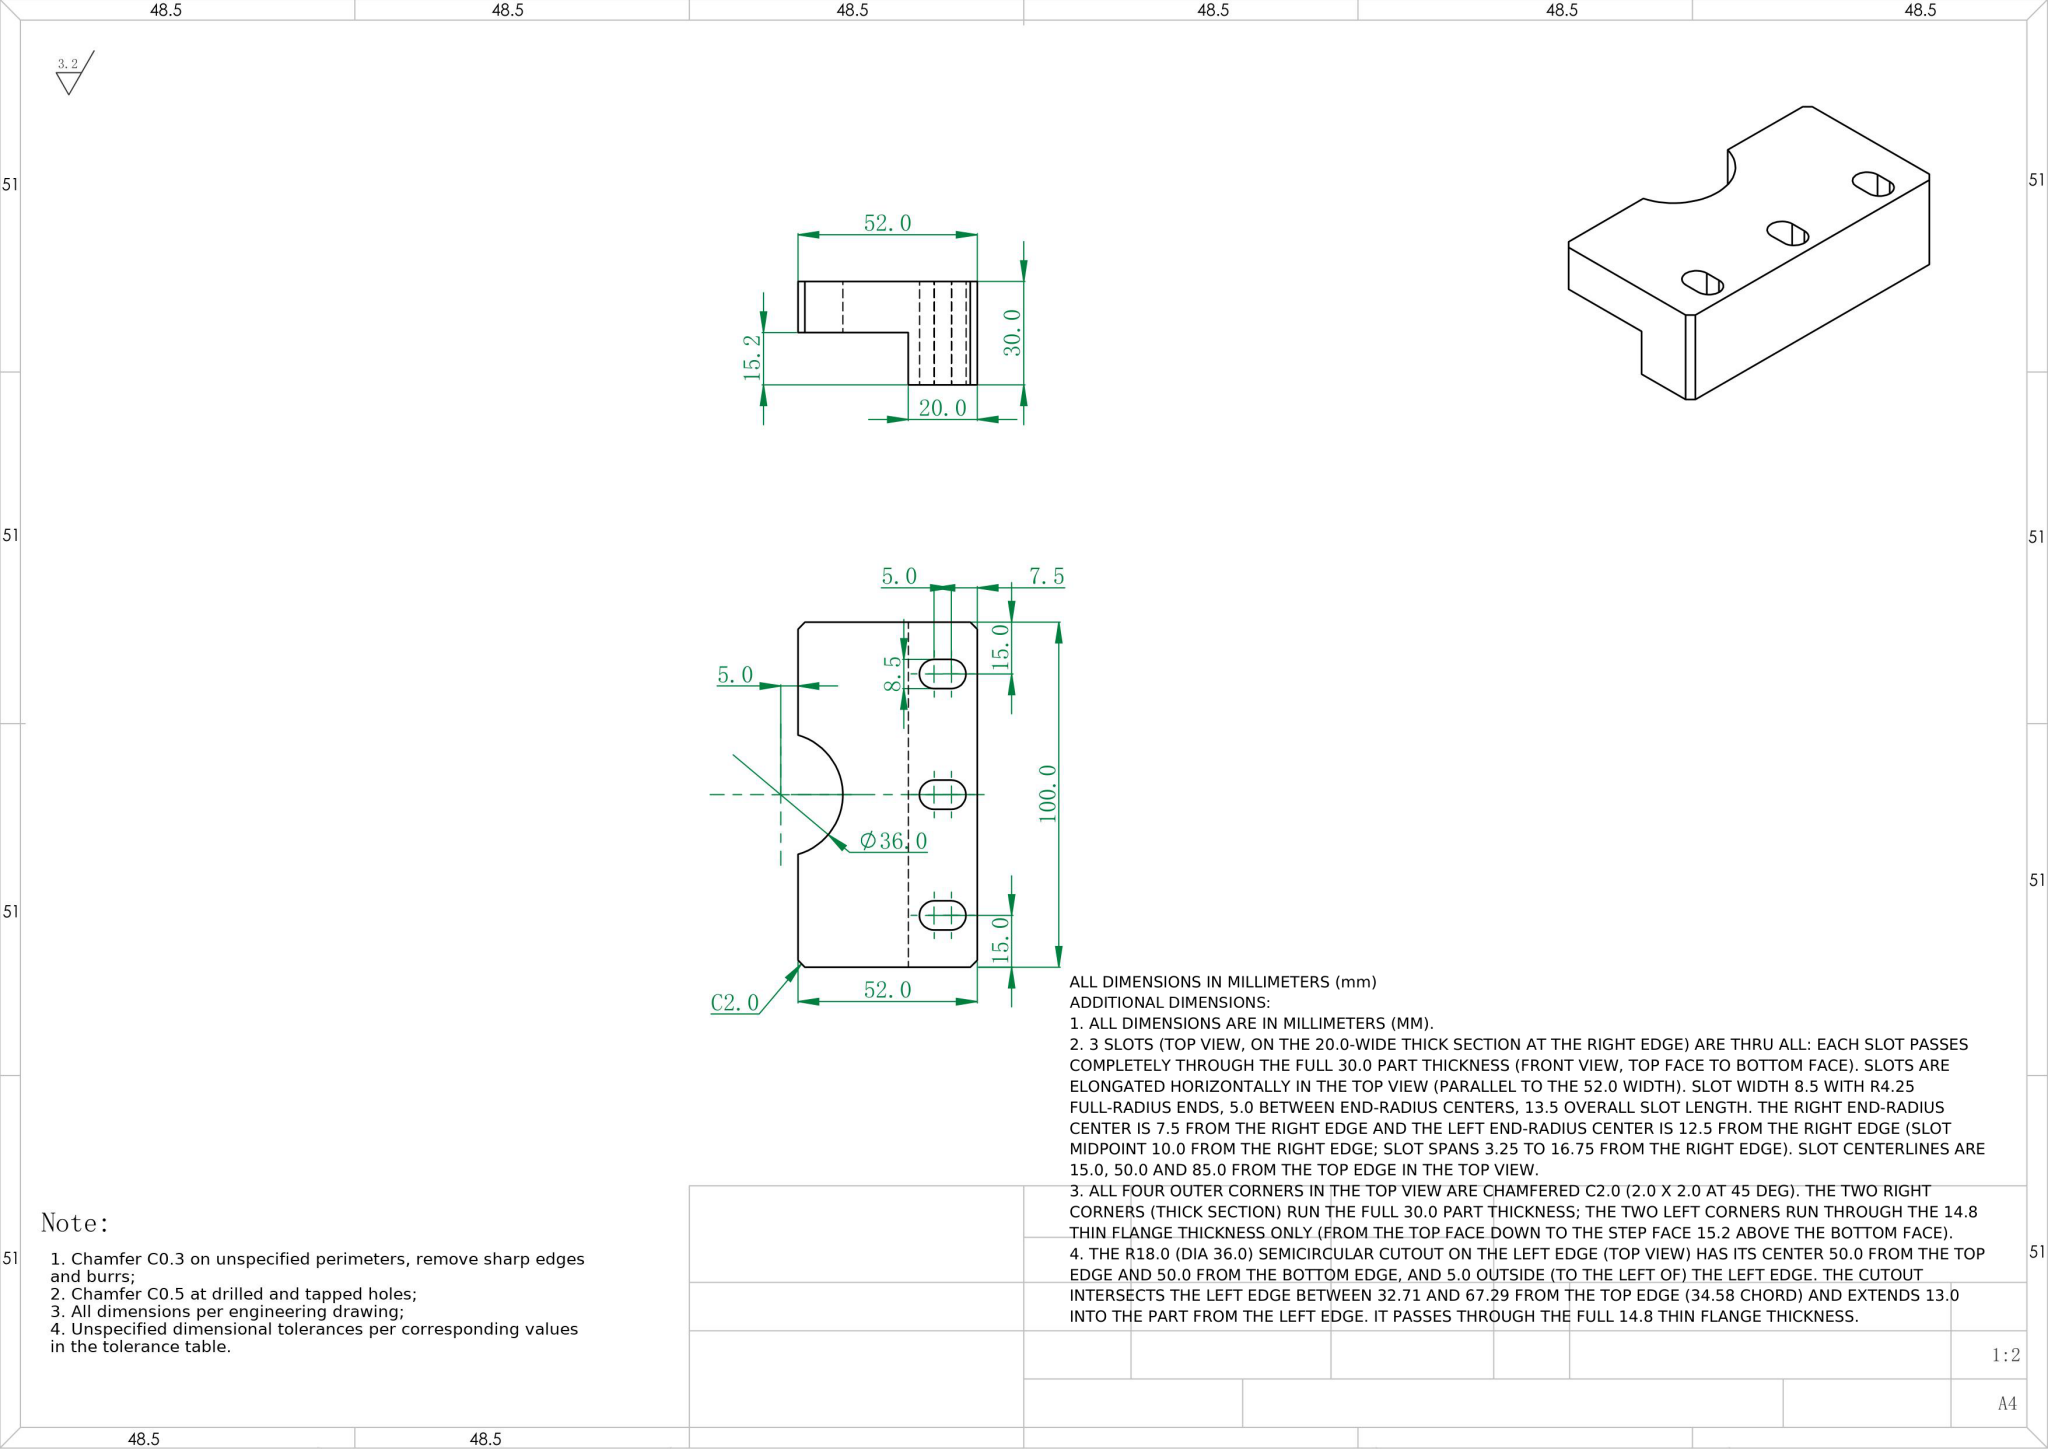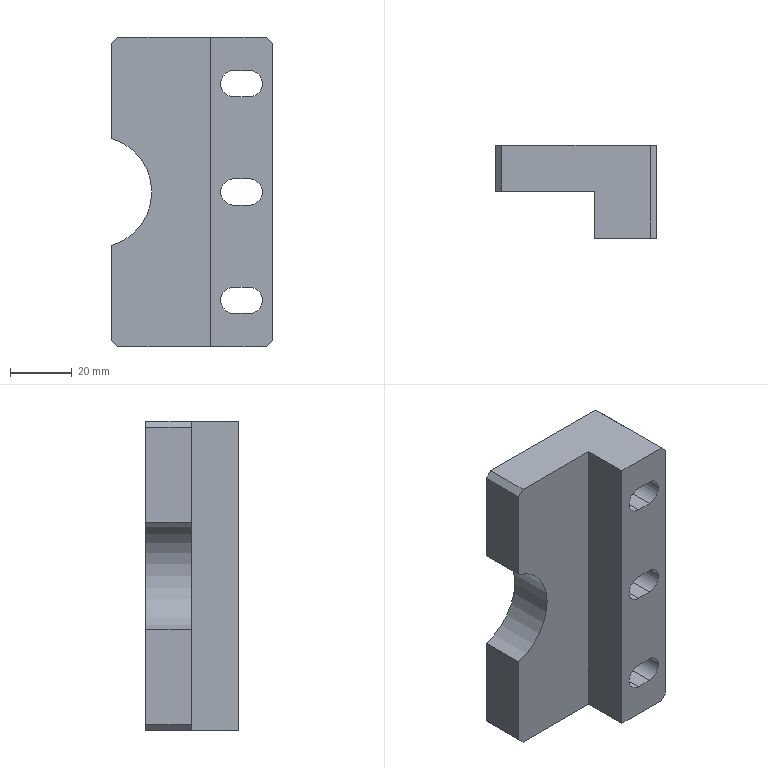Part | NX | mm | Notched Three-Bore Vertical Block | 1 solid | 26 faces | box 52 x 30 x 100 mm | volume 93346 mm3 | plane 19 | cylinder 7 | commonest cylinder face diameters 8.5 x6 36 x1
STEP:
#1=COLOUR_RGB('',0.7922,0.8196,0.9333);
#2=FILL_AREA_STYLE_COLOUR('',#1);
#3=FILL_AREA_STYLE('',(#2));
#4=SURFACE_STYLE_FILL_AREA(#3);
#5=SURFACE_SIDE_STYLE('',(#4));
#6=SURFACE_STYLE_USAGE(.BOTH.,#5);
#7=PRESENTATION_STYLE_ASSIGNMENT((#6));
#8=CARTESIAN_POINT('',(-26.,15.,-48.));
#9=VERTEX_POINT('',#8);
#10=CARTESIAN_POINT('',(-26.,15.,-17.292));
#11=VERTEX_POINT('',#10);
#12=CARTESIAN_POINT('',(-26.,15.,50.));
#13=DIRECTION('',(0.,0.,1.));
#14=VECTOR('',#13,1000.);
#15=LINE('',#12,#14);
#16=EDGE_CURVE('',#9,#11,#15,.T.);
#17=ORIENTED_EDGE('',*,*,#16,.F.);
#18=CARTESIAN_POINT('',(-26.,0.2,-48.));
#19=VERTEX_POINT('',#18);
#20=CARTESIAN_POINT('',(-26.,15.,-48.));
#21=DIRECTION('',(0.,-1.,0.));
#22=VECTOR('',#21,1000.);
#23=LINE('',#20,#22);
#24=EDGE_CURVE('',#9,#19,#23,.T.);
#25=ORIENTED_EDGE('',*,*,#24,.T.);
#26=CARTESIAN_POINT('',(-26.,0.2,-17.292));
#27=VERTEX_POINT('',#26);
#28=CARTESIAN_POINT('',(-26.,0.2,50.));
#29=DIRECTION('',(0.,0.,1.));
#30=VECTOR('',#29,1000.);
#31=LINE('',#28,#30);
#32=EDGE_CURVE('',#19,#27,#31,.T.);
#33=ORIENTED_EDGE('',*,*,#32,.T.);
#34=CARTESIAN_POINT('',(-26.,-15.,-17.292));
#35=DIRECTION('',(0.,1.,0.));
#36=VECTOR('',#35,1000.);
#37=LINE('',#34,#36);
#38=EDGE_CURVE('',#27,#11,#37,.T.);
#39=ORIENTED_EDGE('',*,*,#38,.T.);
#40=EDGE_LOOP('',(#17,#25,#33,#39));
#41=FACE_OUTER_BOUND('',#40,.T.);
#42=CARTESIAN_POINT('',(-26.,15.,50.));
#43=DIRECTION('',(1.,0.,0.));
#44=DIRECTION('',(0.,0.,-1.));
#45=AXIS2_PLACEMENT_3D('',#42,#43,#44);
#46=PLANE('',#45);
#47=ADVANCED_FACE('',(#41),#46,.F.);
#48=CARTESIAN_POINT('',(26.,-15.,48.));
#49=VERTEX_POINT('',#48);
#50=CARTESIAN_POINT('',(26.,-15.,-48.));
#51=VERTEX_POINT('',#50);
#52=CARTESIAN_POINT('',(26.,-15.,50.));
#53=DIRECTION('',(0.,0.,-1.));
#54=VECTOR('',#53,1000.);
#55=LINE('',#52,#54);
#56=EDGE_CURVE('',#49,#51,#55,.T.);
#57=ORIENTED_EDGE('',*,*,#56,.T.);
#58=CARTESIAN_POINT('',(26.,15.,-48.));
#59=VERTEX_POINT('',#58);
#60=CARTESIAN_POINT('',(26.,15.,-48.));
#61=DIRECTION('',(0.,1.,0.));
#62=VECTOR('',#61,1000.);
#63=LINE('',#60,#62);
#64=EDGE_CURVE('',#51,#59,#63,.T.);
#65=ORIENTED_EDGE('',*,*,#64,.T.);
#66=CARTESIAN_POINT('',(26.,15.,48.));
#67=VERTEX_POINT('',#66);
#68=CARTESIAN_POINT('',(26.,15.,50.));
#69=DIRECTION('',(0.,0.,-1.));
#70=VECTOR('',#69,1000.);
#71=LINE('',#68,#70);
#72=EDGE_CURVE('',#67,#59,#71,.T.);
#73=ORIENTED_EDGE('',*,*,#72,.F.);
#74=CARTESIAN_POINT('',(26.,15.,48.));
#75=DIRECTION('',(0.,-1.,0.));
#76=VECTOR('',#75,1000.);
#77=LINE('',#74,#76);
#78=EDGE_CURVE('',#67,#49,#77,.T.);
#79=ORIENTED_EDGE('',*,*,#78,.T.);
#80=EDGE_LOOP('',(#57,#65,#73,#79));
#81=FACE_OUTER_BOUND('',#80,.T.);
#82=CARTESIAN_POINT('',(26.,15.,50.));
#83=DIRECTION('',(-1.,0.,0.));
#84=DIRECTION('',(0.,0.,1.));
#85=AXIS2_PLACEMENT_3D('',#82,#83,#84);
#86=PLANE('',#85);
#87=ADVANCED_FACE('',(#81),#86,.F.);
#88=CARTESIAN_POINT('',(24.,15.,-50.));
#89=VERTEX_POINT('',#88);
#90=CARTESIAN_POINT('',(-24.,15.,-50.));
#91=VERTEX_POINT('',#90);
#92=CARTESIAN_POINT('',(-26.,15.,-50.));
#93=DIRECTION('',(-1.,0.,0.));
#94=VECTOR('',#93,1000.);
#95=LINE('',#92,#94);
#96=EDGE_CURVE('',#89,#91,#95,.T.);
#97=ORIENTED_EDGE('',*,*,#96,.F.);
#98=CARTESIAN_POINT('',(24.,-15.,-50.));
#99=VERTEX_POINT('',#98);
#100=CARTESIAN_POINT('',(24.,15.,-50.));
#101=DIRECTION('',(0.,-1.,0.));
#102=VECTOR('',#101,1000.);
#103=LINE('',#100,#102);
#104=EDGE_CURVE('',#89,#99,#103,.T.);
#105=ORIENTED_EDGE('',*,*,#104,.T.);
#106=CARTESIAN_POINT('',(6.,-15.,-50.));
#107=VERTEX_POINT('',#106);
#108=CARTESIAN_POINT('',(-26.,-15.,-50.));
#109=DIRECTION('',(-1.,0.,0.));
#110=VECTOR('',#109,1000.);
#111=LINE('',#108,#110);
#112=EDGE_CURVE('',#99,#107,#111,.T.);
#113=ORIENTED_EDGE('',*,*,#112,.T.);
#114=CARTESIAN_POINT('',(6.,0.2,-50.));
#115=VERTEX_POINT('',#114);
#116=CARTESIAN_POINT('',(6.,-30.2,-50.));
#117=DIRECTION('',(0.,1.,0.));
#118=VECTOR('',#117,1000.);
#119=LINE('',#116,#118);
#120=EDGE_CURVE('',#107,#115,#119,.T.);
#121=ORIENTED_EDGE('',*,*,#120,.T.);
#122=CARTESIAN_POINT('',(-24.,0.2,-50.));
#123=VERTEX_POINT('',#122);
#124=CARTESIAN_POINT('',(-58.,0.2,-50.));
#125=DIRECTION('',(-1.,0.,0.));
#126=VECTOR('',#125,1000.);
#127=LINE('',#124,#126);
#128=EDGE_CURVE('',#115,#123,#127,.T.);
#129=ORIENTED_EDGE('',*,*,#128,.T.);
#130=CARTESIAN_POINT('',(-24.,15.,-50.));
#131=DIRECTION('',(0.,1.,0.));
#132=VECTOR('',#131,1000.);
#133=LINE('',#130,#132);
#134=EDGE_CURVE('',#123,#91,#133,.T.);
#135=ORIENTED_EDGE('',*,*,#134,.T.);
#136=EDGE_LOOP('',(#97,#105,#113,#121,#129,#135));
#137=FACE_OUTER_BOUND('',#136,.T.);
#138=CARTESIAN_POINT('',(-26.,15.,-50.));
#139=DIRECTION('',(0.,0.,1.));
#140=DIRECTION('',(1.,0.,0.));
#141=AXIS2_PLACEMENT_3D('',#138,#139,#140);
#142=PLANE('',#141);
#143=ADVANCED_FACE('',(#137),#142,.F.);
#144=CARTESIAN_POINT('',(-26.,0.2,17.292));
#145=VERTEX_POINT('',#144);
#146=CARTESIAN_POINT('',(-26.,0.2,48.));
#147=VERTEX_POINT('',#146);
#148=CARTESIAN_POINT('',(-26.,0.2,50.));
#149=DIRECTION('',(0.,0.,1.));
#150=VECTOR('',#149,1000.);
#151=LINE('',#148,#150);
#152=EDGE_CURVE('',#145,#147,#151,.T.);
#153=ORIENTED_EDGE('',*,*,#152,.T.);
#154=CARTESIAN_POINT('',(-26.,15.,48.));
#155=VERTEX_POINT('',#154);
#156=CARTESIAN_POINT('',(-26.,15.,48.));
#157=DIRECTION('',(0.,1.,0.));
#158=VECTOR('',#157,1000.);
#159=LINE('',#156,#158);
#160=EDGE_CURVE('',#147,#155,#159,.T.);
#161=ORIENTED_EDGE('',*,*,#160,.T.);
#162=CARTESIAN_POINT('',(-26.,15.,17.292));
#163=VERTEX_POINT('',#162);
#164=CARTESIAN_POINT('',(-26.,15.,50.));
#165=DIRECTION('',(0.,0.,1.));
#166=VECTOR('',#165,1000.);
#167=LINE('',#164,#166);
#168=EDGE_CURVE('',#163,#155,#167,.T.);
#169=ORIENTED_EDGE('',*,*,#168,.F.);
#170=CARTESIAN_POINT('',(-26.,-15.,17.292));
#171=DIRECTION('',(0.,-1.,0.));
#172=VECTOR('',#171,1000.);
#173=LINE('',#170,#172);
#174=EDGE_CURVE('',#163,#145,#173,.T.);
#175=ORIENTED_EDGE('',*,*,#174,.T.);
#176=EDGE_LOOP('',(#153,#161,#169,#175));
#177=FACE_OUTER_BOUND('',#176,.T.);
#178=CARTESIAN_POINT('',(-26.,15.,50.));
#179=DIRECTION('',(1.,0.,0.));
#180=DIRECTION('',(0.,0.,-1.));
#181=AXIS2_PLACEMENT_3D('',#178,#179,#180);
#182=PLANE('',#181);
#183=ADVANCED_FACE('',(#177),#182,.F.);
#184=CARTESIAN_POINT('',(6.,-15.,50.));
#185=VERTEX_POINT('',#184);
#186=CARTESIAN_POINT('',(24.,-15.,50.));
#187=VERTEX_POINT('',#186);
#188=CARTESIAN_POINT('',(-26.,-15.,50.));
#189=DIRECTION('',(1.,0.,0.));
#190=VECTOR('',#189,1000.);
#191=LINE('',#188,#190);
#192=EDGE_CURVE('',#185,#187,#191,.T.);
#193=ORIENTED_EDGE('',*,*,#192,.T.);
#194=CARTESIAN_POINT('',(24.,15.,50.));
#195=VERTEX_POINT('',#194);
#196=CARTESIAN_POINT('',(24.,15.,50.));
#197=DIRECTION('',(0.,1.,0.));
#198=VECTOR('',#197,1000.);
#199=LINE('',#196,#198);
#200=EDGE_CURVE('',#187,#195,#199,.T.);
#201=ORIENTED_EDGE('',*,*,#200,.T.);
#202=CARTESIAN_POINT('',(-24.,15.,50.));
#203=VERTEX_POINT('',#202);
#204=CARTESIAN_POINT('',(-26.,15.,50.));
#205=DIRECTION('',(1.,0.,0.));
#206=VECTOR('',#205,1000.);
#207=LINE('',#204,#206);
#208=EDGE_CURVE('',#203,#195,#207,.T.);
#209=ORIENTED_EDGE('',*,*,#208,.F.);
#210=CARTESIAN_POINT('',(-24.,0.2,50.));
#211=VERTEX_POINT('',#210);
#212=CARTESIAN_POINT('',(-24.,15.,50.));
#213=DIRECTION('',(0.,-1.,0.));
#214=VECTOR('',#213,1000.);
#215=LINE('',#212,#214);
#216=EDGE_CURVE('',#203,#211,#215,.T.);
#217=ORIENTED_EDGE('',*,*,#216,.T.);
#218=CARTESIAN_POINT('',(6.,0.2,50.));
#219=VERTEX_POINT('',#218);
#220=CARTESIAN_POINT('',(-58.,0.2,50.));
#221=DIRECTION('',(-1.,0.,0.));
#222=VECTOR('',#221,1000.);
#223=LINE('',#220,#222);
#224=EDGE_CURVE('',#219,#211,#223,.T.);
#225=ORIENTED_EDGE('',*,*,#224,.F.);
#226=CARTESIAN_POINT('',(6.,-30.2,50.));
#227=DIRECTION('',(0.,1.,0.));
#228=VECTOR('',#227,1000.);
#229=LINE('',#226,#228);
#230=EDGE_CURVE('',#185,#219,#229,.T.);
#231=ORIENTED_EDGE('',*,*,#230,.F.);
#232=EDGE_LOOP('',(#193,#201,#209,#217,#225,#231));
#233=FACE_OUTER_BOUND('',#232,.T.);
#234=CARTESIAN_POINT('',(-26.,15.,50.));
#235=DIRECTION('',(0.,0.,-1.));
#236=DIRECTION('',(-1.,0.,0.));
#237=AXIS2_PLACEMENT_3D('',#234,#235,#236);
#238=PLANE('',#237);
#239=ADVANCED_FACE('',(#233),#238,.F.);
#240=CARTESIAN_POINT('',(13.5,15.,4.25));
#241=VERTEX_POINT('',#240);
#242=CARTESIAN_POINT('',(18.5,15.,4.25));
#243=VERTEX_POINT('',#242);
#244=CARTESIAN_POINT('',(13.5,15.,4.25));
#245=DIRECTION('',(1.,0.,-0.));
#246=VECTOR('',#245,1000.);
#247=LINE('',#244,#246);
#248=EDGE_CURVE('',#241,#243,#247,.T.);
#249=ORIENTED_EDGE('',*,*,#248,.F.);
#250=CARTESIAN_POINT('',(13.5,15.,-4.25));
#251=VERTEX_POINT('',#250);
#252=CARTESIAN_POINT('',(13.5,15.,0.));
#253=DIRECTION('',(0.,1.,0.));
#254=DIRECTION('',(0.,0.,1.));
#255=AXIS2_PLACEMENT_3D('',#252,#253,#254);
#256=CIRCLE('',#255,4.25);
#257=EDGE_CURVE('',#251,#241,#256,.T.);
#258=ORIENTED_EDGE('',*,*,#257,.F.);
#259=CARTESIAN_POINT('',(18.5,15.,-4.25));
#260=VERTEX_POINT('',#259);
#261=CARTESIAN_POINT('',(13.5,15.,-4.25));
#262=DIRECTION('',(-1.,0.,0.));
#263=VECTOR('',#262,1000.);
#264=LINE('',#261,#263);
#265=EDGE_CURVE('',#260,#251,#264,.T.);
#266=ORIENTED_EDGE('',*,*,#265,.F.);
#267=CARTESIAN_POINT('',(18.5,15.,-0.));
#268=DIRECTION('',(0.,1.,0.));
#269=DIRECTION('',(0.,0.,1.));
#270=AXIS2_PLACEMENT_3D('',#267,#268,#269);
#271=CIRCLE('',#270,4.25);
#272=EDGE_CURVE('',#243,#260,#271,.T.);
#273=ORIENTED_EDGE('',*,*,#272,.F.);
#274=EDGE_LOOP('',(#249,#258,#266,#273));
#275=FACE_BOUND('',#274,.T.);
#276=CARTESIAN_POINT('',(13.5,15.,39.25));
#277=VERTEX_POINT('',#276);
#278=CARTESIAN_POINT('',(18.5,15.,39.25));
#279=VERTEX_POINT('',#278);
#280=CARTESIAN_POINT('',(13.5,15.,39.25));
#281=DIRECTION('',(1.,0.,0.));
#282=VECTOR('',#281,1000.);
#283=LINE('',#280,#282);
#284=EDGE_CURVE('',#277,#279,#283,.T.);
#285=ORIENTED_EDGE('',*,*,#284,.F.);
#286=CARTESIAN_POINT('',(13.5,15.,30.75));
#287=VERTEX_POINT('',#286);
#288=CARTESIAN_POINT('',(13.5,15.,35.));
#289=DIRECTION('',(0.,1.,0.));
#290=DIRECTION('',(0.,0.,1.));
#291=AXIS2_PLACEMENT_3D('',#288,#289,#290);
#292=CIRCLE('',#291,4.25);
#293=EDGE_CURVE('',#287,#277,#292,.T.);
#294=ORIENTED_EDGE('',*,*,#293,.F.);
#295=CARTESIAN_POINT('',(18.5,15.,30.75));
#296=VERTEX_POINT('',#295);
#297=CARTESIAN_POINT('',(13.5,15.,30.75));
#298=DIRECTION('',(-1.,0.,0.));
#299=VECTOR('',#298,1000.);
#300=LINE('',#297,#299);
#301=EDGE_CURVE('',#296,#287,#300,.T.);
#302=ORIENTED_EDGE('',*,*,#301,.F.);
#303=CARTESIAN_POINT('',(18.5,15.,35.));
#304=DIRECTION('',(0.,1.,0.));
#305=DIRECTION('',(0.,0.,1.));
#306=AXIS2_PLACEMENT_3D('',#303,#304,#305);
#307=CIRCLE('',#306,4.25);
#308=EDGE_CURVE('',#279,#296,#307,.T.);
#309=ORIENTED_EDGE('',*,*,#308,.F.);
#310=EDGE_LOOP('',(#285,#294,#302,#309));
#311=FACE_BOUND('',#310,.T.);
#312=CARTESIAN_POINT('',(13.5,15.,-30.75));
#313=VERTEX_POINT('',#312);
#314=CARTESIAN_POINT('',(18.5,15.,-30.75));
#315=VERTEX_POINT('',#314);
#316=CARTESIAN_POINT('',(13.5,15.,-30.75));
#317=DIRECTION('',(1.,0.,0.));
#318=VECTOR('',#317,1000.);
#319=LINE('',#316,#318);
#320=EDGE_CURVE('',#313,#315,#319,.T.);
#321=ORIENTED_EDGE('',*,*,#320,.F.);
#322=CARTESIAN_POINT('',(13.5,15.,-39.25));
#323=VERTEX_POINT('',#322);
#324=CARTESIAN_POINT('',(13.5,15.,-35.));
#325=DIRECTION('',(0.,1.,0.));
#326=DIRECTION('',(0.,0.,1.));
#327=AXIS2_PLACEMENT_3D('',#324,#325,#326);
#328=CIRCLE('',#327,4.25);
#329=EDGE_CURVE('',#323,#313,#328,.T.);
#330=ORIENTED_EDGE('',*,*,#329,.F.);
#331=CARTESIAN_POINT('',(18.5,15.,-39.25));
#332=VERTEX_POINT('',#331);
#333=CARTESIAN_POINT('',(13.5,15.,-39.25));
#334=DIRECTION('',(-1.,0.,0.));
#335=VECTOR('',#334,1000.);
#336=LINE('',#333,#335);
#337=EDGE_CURVE('',#332,#323,#336,.T.);
#338=ORIENTED_EDGE('',*,*,#337,.F.);
#339=CARTESIAN_POINT('',(18.5,15.,-35.));
#340=DIRECTION('',(0.,1.,0.));
#341=DIRECTION('',(0.,0.,1.));
#342=AXIS2_PLACEMENT_3D('',#339,#340,#341);
#343=CIRCLE('',#342,4.25);
#344=EDGE_CURVE('',#315,#332,#343,.T.);
#345=ORIENTED_EDGE('',*,*,#344,.F.);
#346=EDGE_LOOP('',(#321,#330,#338,#345));
#347=FACE_BOUND('',#346,.T.);
#348=ORIENTED_EDGE('',*,*,#72,.T.);
#349=CARTESIAN_POINT('',(24.,15.,-50.));
#350=DIRECTION('',(-0.7071,0.,-0.7071));
#351=VECTOR('',#350,1000.);
#352=LINE('',#349,#351);
#353=EDGE_CURVE('',#59,#89,#352,.T.);
#354=ORIENTED_EDGE('',*,*,#353,.T.);
#355=ORIENTED_EDGE('',*,*,#96,.T.);
#356=CARTESIAN_POINT('',(-26.,15.,-48.));
#357=DIRECTION('',(-0.7071,0.,0.7071));
#358=VECTOR('',#357,1000.);
#359=LINE('',#356,#358);
#360=EDGE_CURVE('',#91,#9,#359,.T.);
#361=ORIENTED_EDGE('',*,*,#360,.T.);
#362=ORIENTED_EDGE('',*,*,#16,.T.);
#363=CARTESIAN_POINT('',(-31.,15.,0.));
#364=DIRECTION('',(0.,1.,0.));
#365=DIRECTION('',(0.,0.,1.));
#366=AXIS2_PLACEMENT_3D('',#363,#364,#365);
#367=CIRCLE('',#366,18.);
#368=EDGE_CURVE('',#163,#11,#367,.T.);
#369=ORIENTED_EDGE('',*,*,#368,.F.);
#370=ORIENTED_EDGE('',*,*,#168,.T.);
#371=CARTESIAN_POINT('',(-24.,15.,50.));
#372=DIRECTION('',(0.7071,0.,0.7071));
#373=VECTOR('',#372,1000.);
#374=LINE('',#371,#373);
#375=EDGE_CURVE('',#155,#203,#374,.T.);
#376=ORIENTED_EDGE('',*,*,#375,.T.);
#377=ORIENTED_EDGE('',*,*,#208,.T.);
#378=CARTESIAN_POINT('',(26.,15.,48.));
#379=DIRECTION('',(0.7071,0.,-0.7071));
#380=VECTOR('',#379,1000.);
#381=LINE('',#378,#380);
#382=EDGE_CURVE('',#195,#67,#381,.T.);
#383=ORIENTED_EDGE('',*,*,#382,.T.);
#384=EDGE_LOOP('',(#348,#354,#355,#361,#362,#369,#370,#376,#377,#383));
#385=FACE_OUTER_BOUND('',#384,.T.);
#386=CARTESIAN_POINT('',(0.,15.,0.));
#387=DIRECTION('',(0.,-1.,0.));
#388=DIRECTION('',(0.,0.,-1.));
#389=AXIS2_PLACEMENT_3D('',#386,#387,#388);
#390=PLANE('',#389);
#391=ADVANCED_FACE('',(#275,#311,#347,#385),#390,.F.);
#392=CARTESIAN_POINT('',(13.5,-15.,-4.25));
#393=VERTEX_POINT('',#392);
#394=CARTESIAN_POINT('',(13.5,-15.,4.25));
#395=VERTEX_POINT('',#394);
#396=CARTESIAN_POINT('',(13.5,-15.,0.));
#397=DIRECTION('',(0.,1.,0.));
#398=DIRECTION('',(0.,0.,1.));
#399=AXIS2_PLACEMENT_3D('',#396,#397,#398);
#400=CIRCLE('',#399,4.25);
#401=EDGE_CURVE('',#393,#395,#400,.T.);
#402=ORIENTED_EDGE('',*,*,#401,.T.);
#403=CARTESIAN_POINT('',(18.5,-15.,4.25));
#404=VERTEX_POINT('',#403);
#405=CARTESIAN_POINT('',(13.5,-15.,4.25));
#406=DIRECTION('',(1.,0.,-0.));
#407=VECTOR('',#406,1000.);
#408=LINE('',#405,#407);
#409=EDGE_CURVE('',#395,#404,#408,.T.);
#410=ORIENTED_EDGE('',*,*,#409,.T.);
#411=CARTESIAN_POINT('',(18.5,-15.,-4.25));
#412=VERTEX_POINT('',#411);
#413=CARTESIAN_POINT('',(18.5,-15.,-0.));
#414=DIRECTION('',(0.,1.,0.));
#415=DIRECTION('',(0.,0.,1.));
#416=AXIS2_PLACEMENT_3D('',#413,#414,#415);
#417=CIRCLE('',#416,4.25);
#418=EDGE_CURVE('',#404,#412,#417,.T.);
#419=ORIENTED_EDGE('',*,*,#418,.T.);
#420=CARTESIAN_POINT('',(13.5,-15.,-4.25));
#421=DIRECTION('',(-1.,0.,0.));
#422=VECTOR('',#421,1000.);
#423=LINE('',#420,#422);
#424=EDGE_CURVE('',#412,#393,#423,.T.);
#425=ORIENTED_EDGE('',*,*,#424,.T.);
#426=EDGE_LOOP('',(#402,#410,#419,#425));
#427=FACE_BOUND('',#426,.T.);
#428=CARTESIAN_POINT('',(13.5,-15.,30.75));
#429=VERTEX_POINT('',#428);
#430=CARTESIAN_POINT('',(13.5,-15.,39.25));
#431=VERTEX_POINT('',#430);
#432=CARTESIAN_POINT('',(13.5,-15.,35.));
#433=DIRECTION('',(0.,1.,0.));
#434=DIRECTION('',(0.,0.,1.));
#435=AXIS2_PLACEMENT_3D('',#432,#433,#434);
#436=CIRCLE('',#435,4.25);
#437=EDGE_CURVE('',#429,#431,#436,.T.);
#438=ORIENTED_EDGE('',*,*,#437,.T.);
#439=CARTESIAN_POINT('',(18.5,-15.,39.25));
#440=VERTEX_POINT('',#439);
#441=CARTESIAN_POINT('',(13.5,-15.,39.25));
#442=DIRECTION('',(1.,0.,0.));
#443=VECTOR('',#442,1000.);
#444=LINE('',#441,#443);
#445=EDGE_CURVE('',#431,#440,#444,.T.);
#446=ORIENTED_EDGE('',*,*,#445,.T.);
#447=CARTESIAN_POINT('',(18.5,-15.,30.75));
#448=VERTEX_POINT('',#447);
#449=CARTESIAN_POINT('',(18.5,-15.,35.));
#450=DIRECTION('',(0.,1.,0.));
#451=DIRECTION('',(0.,0.,1.));
#452=AXIS2_PLACEMENT_3D('',#449,#450,#451);
#453=CIRCLE('',#452,4.25);
#454=EDGE_CURVE('',#440,#448,#453,.T.);
#455=ORIENTED_EDGE('',*,*,#454,.T.);
#456=CARTESIAN_POINT('',(13.5,-15.,30.75));
#457=DIRECTION('',(-1.,0.,0.));
#458=VECTOR('',#457,1000.);
#459=LINE('',#456,#458);
#460=EDGE_CURVE('',#448,#429,#459,.T.);
#461=ORIENTED_EDGE('',*,*,#460,.T.);
#462=EDGE_LOOP('',(#438,#446,#455,#461));
#463=FACE_BOUND('',#462,.T.);
#464=CARTESIAN_POINT('',(13.5,-15.,-39.25));
#465=VERTEX_POINT('',#464);
#466=CARTESIAN_POINT('',(13.5,-15.,-30.75));
#467=VERTEX_POINT('',#466);
#468=CARTESIAN_POINT('',(13.5,-15.,-35.));
#469=DIRECTION('',(0.,1.,0.));
#470=DIRECTION('',(0.,0.,1.));
#471=AXIS2_PLACEMENT_3D('',#468,#469,#470);
#472=CIRCLE('',#471,4.25);
#473=EDGE_CURVE('',#465,#467,#472,.T.);
#474=ORIENTED_EDGE('',*,*,#473,.T.);
#475=CARTESIAN_POINT('',(18.5,-15.,-30.75));
#476=VERTEX_POINT('',#475);
#477=CARTESIAN_POINT('',(13.5,-15.,-30.75));
#478=DIRECTION('',(1.,0.,0.));
#479=VECTOR('',#478,1000.);
#480=LINE('',#477,#479);
#481=EDGE_CURVE('',#467,#476,#480,.T.);
#482=ORIENTED_EDGE('',*,*,#481,.T.);
#483=CARTESIAN_POINT('',(18.5,-15.,-39.25));
#484=VERTEX_POINT('',#483);
#485=CARTESIAN_POINT('',(18.5,-15.,-35.));
#486=DIRECTION('',(0.,1.,0.));
#487=DIRECTION('',(0.,0.,1.));
#488=AXIS2_PLACEMENT_3D('',#485,#486,#487);
#489=CIRCLE('',#488,4.25);
#490=EDGE_CURVE('',#476,#484,#489,.T.);
#491=ORIENTED_EDGE('',*,*,#490,.T.);
#492=CARTESIAN_POINT('',(13.5,-15.,-39.25));
#493=DIRECTION('',(-1.,0.,0.));
#494=VECTOR('',#493,1000.);
#495=LINE('',#492,#494);
#496=EDGE_CURVE('',#484,#465,#495,.T.);
#497=ORIENTED_EDGE('',*,*,#496,.T.);
#498=EDGE_LOOP('',(#474,#482,#491,#497));
#499=FACE_BOUND('',#498,.T.);
#500=ORIENTED_EDGE('',*,*,#112,.F.);
#501=CARTESIAN_POINT('',(37.,-15.,-37.));
#502=DIRECTION('',(0.7071,0.,0.7071));
#503=VECTOR('',#502,1000.);
#504=LINE('',#501,#503);
#505=EDGE_CURVE('',#99,#51,#504,.T.);
#506=ORIENTED_EDGE('',*,*,#505,.T.);
#507=ORIENTED_EDGE('',*,*,#56,.F.);
#508=CARTESIAN_POINT('',(37.,-15.,37.));
#509=DIRECTION('',(-0.7071,0.,0.7071));
#510=VECTOR('',#509,1000.);
#511=LINE('',#508,#510);
#512=EDGE_CURVE('',#49,#187,#511,.T.);
#513=ORIENTED_EDGE('',*,*,#512,.T.);
#514=ORIENTED_EDGE('',*,*,#192,.F.);
#515=CARTESIAN_POINT('',(6.,-15.,0.));
#516=DIRECTION('',(0.,0.,1.));
#517=VECTOR('',#516,1000.);
#518=LINE('',#515,#517);
#519=EDGE_CURVE('',#107,#185,#518,.T.);
#520=ORIENTED_EDGE('',*,*,#519,.F.);
#521=EDGE_LOOP('',(#500,#506,#507,#513,#514,#520));
#522=FACE_OUTER_BOUND('',#521,.T.);
#523=CARTESIAN_POINT('',(0.,-15.,0.));
#524=DIRECTION('',(0.,-1.,0.));
#525=DIRECTION('',(0.,0.,-1.));
#526=AXIS2_PLACEMENT_3D('',#523,#524,#525);
#527=PLANE('',#526);
#528=ADVANCED_FACE('',(#427,#463,#499,#522),#527,.T.);
#529=ORIENTED_EDGE('',*,*,#32,.F.);
#530=CARTESIAN_POINT('',(-26.,0.2,-48.));
#531=DIRECTION('',(0.7071,0.,-0.7071));
#532=VECTOR('',#531,1000.);
#533=LINE('',#530,#532);
#534=EDGE_CURVE('',#19,#123,#533,.T.);
#535=ORIENTED_EDGE('',*,*,#534,.T.);
#536=ORIENTED_EDGE('',*,*,#128,.F.);
#537=CARTESIAN_POINT('',(6.,0.2,-50.));
#538=DIRECTION('',(0.,0.,1.));
#539=VECTOR('',#538,1000.);
#540=LINE('',#537,#539);
#541=EDGE_CURVE('',#115,#219,#540,.T.);
#542=ORIENTED_EDGE('',*,*,#541,.T.);
#543=ORIENTED_EDGE('',*,*,#224,.T.);
#544=CARTESIAN_POINT('',(-24.,0.2,50.));
#545=DIRECTION('',(-0.7071,0.,-0.7071));
#546=VECTOR('',#545,1000.);
#547=LINE('',#544,#546);
#548=EDGE_CURVE('',#211,#147,#547,.T.);
#549=ORIENTED_EDGE('',*,*,#548,.T.);
#550=ORIENTED_EDGE('',*,*,#152,.F.);
#551=CARTESIAN_POINT('',(-31.,0.2,0.));
#552=DIRECTION('',(0.,1.,0.));
#553=DIRECTION('',(0.,0.,1.));
#554=AXIS2_PLACEMENT_3D('',#551,#552,#553);
#555=CIRCLE('',#554,18.);
#556=EDGE_CURVE('',#145,#27,#555,.T.);
#557=ORIENTED_EDGE('',*,*,#556,.T.);
#558=EDGE_LOOP('',(#529,#535,#536,#542,#543,#549,#550,#557));
#559=FACE_OUTER_BOUND('',#558,.T.);
#560=CARTESIAN_POINT('',(-58.,0.2,-50.));
#561=DIRECTION('',(0.,1.,0.));
#562=DIRECTION('',(0.,0.,1.));
#563=AXIS2_PLACEMENT_3D('',#560,#561,#562);
#564=PLANE('',#563);
#565=ADVANCED_FACE('',(#559),#564,.F.);
#566=ORIENTED_EDGE('',*,*,#519,.T.);
#567=ORIENTED_EDGE('',*,*,#230,.T.);
#568=ORIENTED_EDGE('',*,*,#541,.F.);
#569=ORIENTED_EDGE('',*,*,#120,.F.);
#570=EDGE_LOOP('',(#566,#567,#568,#569));
#571=FACE_OUTER_BOUND('',#570,.T.);
#572=CARTESIAN_POINT('',(6.,-30.2,-50.));
#573=DIRECTION('',(1.,0.,0.));
#574=DIRECTION('',(0.,0.,-1.));
#575=AXIS2_PLACEMENT_3D('',#572,#573,#574);
#576=PLANE('',#575);
#577=ADVANCED_FACE('',(#571),#576,.F.);
#578=ORIENTED_EDGE('',*,*,#329,.T.);
#579=CARTESIAN_POINT('',(13.5,-15.,-30.75));
#580=DIRECTION('',(0.,1.,0.));
#581=VECTOR('',#580,1000.);
#582=LINE('',#579,#581);
#583=EDGE_CURVE('',#467,#313,#582,.T.);
#584=ORIENTED_EDGE('',*,*,#583,.F.);
#585=ORIENTED_EDGE('',*,*,#473,.F.);
#586=CARTESIAN_POINT('',(13.5,-15.,-39.25));
#587=DIRECTION('',(0.,1.,0.));
#588=VECTOR('',#587,1000.);
#589=LINE('',#586,#588);
#590=EDGE_CURVE('',#465,#323,#589,.T.);
#591=ORIENTED_EDGE('',*,*,#590,.T.);
#592=EDGE_LOOP('',(#578,#584,#585,#591));
#593=FACE_OUTER_BOUND('',#592,.T.);
#594=CARTESIAN_POINT('',(13.5,-15.,-35.));
#595=DIRECTION('',(0.,1.,0.));
#596=DIRECTION('',(0.,0.,1.));
#597=AXIS2_PLACEMENT_3D('',#594,#595,#596);
#598=CYLINDRICAL_SURFACE('',#597,4.25);
#599=ADVANCED_FACE('',(#593),#598,.F.);
#600=ORIENTED_EDGE('',*,*,#337,.T.);
#601=ORIENTED_EDGE('',*,*,#590,.F.);
#602=ORIENTED_EDGE('',*,*,#496,.F.);
#603=CARTESIAN_POINT('',(18.5,-15.,-39.25));
#604=DIRECTION('',(0.,1.,0.));
#605=VECTOR('',#604,1000.);
#606=LINE('',#603,#605);
#607=EDGE_CURVE('',#484,#332,#606,.T.);
#608=ORIENTED_EDGE('',*,*,#607,.T.);
#609=EDGE_LOOP('',(#600,#601,#602,#608));
#610=FACE_OUTER_BOUND('',#609,.T.);
#611=CARTESIAN_POINT('',(13.5,-15.,-39.25));
#612=DIRECTION('',(0.,0.,-1.));
#613=DIRECTION('',(-1.,0.,0.));
#614=AXIS2_PLACEMENT_3D('',#611,#612,#613);
#615=PLANE('',#614);
#616=ADVANCED_FACE('',(#610),#615,.F.);
#617=ORIENTED_EDGE('',*,*,#344,.T.);
#618=ORIENTED_EDGE('',*,*,#607,.F.);
#619=ORIENTED_EDGE('',*,*,#490,.F.);
#620=CARTESIAN_POINT('',(18.5,-15.,-30.75));
#621=DIRECTION('',(0.,1.,0.));
#622=VECTOR('',#621,1000.);
#623=LINE('',#620,#622);
#624=EDGE_CURVE('',#476,#315,#623,.T.);
#625=ORIENTED_EDGE('',*,*,#624,.T.);
#626=EDGE_LOOP('',(#617,#618,#619,#625));
#627=FACE_OUTER_BOUND('',#626,.T.);
#628=CARTESIAN_POINT('',(18.5,-15.,-35.));
#629=DIRECTION('',(0.,1.,0.));
#630=DIRECTION('',(0.,0.,1.));
#631=AXIS2_PLACEMENT_3D('',#628,#629,#630);
#632=CYLINDRICAL_SURFACE('',#631,4.25);
#633=ADVANCED_FACE('',(#627),#632,.F.);
#634=ORIENTED_EDGE('',*,*,#320,.T.);
#635=ORIENTED_EDGE('',*,*,#624,.F.);
#636=ORIENTED_EDGE('',*,*,#481,.F.);
#637=ORIENTED_EDGE('',*,*,#583,.T.);
#638=EDGE_LOOP('',(#634,#635,#636,#637));
#639=FACE_OUTER_BOUND('',#638,.T.);
#640=CARTESIAN_POINT('',(13.5,-15.,-30.75));
#641=DIRECTION('',(0.,0.,1.));
#642=DIRECTION('',(1.,0.,0.));
#643=AXIS2_PLACEMENT_3D('',#640,#641,#642);
#644=PLANE('',#643);
#645=ADVANCED_FACE('',(#639),#644,.F.);
#646=ORIENTED_EDGE('',*,*,#293,.T.);
#647=CARTESIAN_POINT('',(13.5,-15.,39.25));
#648=DIRECTION('',(0.,1.,0.));
#649=VECTOR('',#648,1000.);
#650=LINE('',#647,#649);
#651=EDGE_CURVE('',#431,#277,#650,.T.);
#652=ORIENTED_EDGE('',*,*,#651,.F.);
#653=ORIENTED_EDGE('',*,*,#437,.F.);
#654=CARTESIAN_POINT('',(13.5,-15.,30.75));
#655=DIRECTION('',(0.,1.,0.));
#656=VECTOR('',#655,1000.);
#657=LINE('',#654,#656);
#658=EDGE_CURVE('',#429,#287,#657,.T.);
#659=ORIENTED_EDGE('',*,*,#658,.T.);
#660=EDGE_LOOP('',(#646,#652,#653,#659));
#661=FACE_OUTER_BOUND('',#660,.T.);
#662=CARTESIAN_POINT('',(13.5,-15.,35.));
#663=DIRECTION('',(0.,1.,0.));
#664=DIRECTION('',(0.,0.,1.));
#665=AXIS2_PLACEMENT_3D('',#662,#663,#664);
#666=CYLINDRICAL_SURFACE('',#665,4.25);
#667=ADVANCED_FACE('',(#661),#666,.F.);
#668=ORIENTED_EDGE('',*,*,#301,.T.);
#669=ORIENTED_EDGE('',*,*,#658,.F.);
#670=ORIENTED_EDGE('',*,*,#460,.F.);
#671=CARTESIAN_POINT('',(18.5,-15.,30.75));
#672=DIRECTION('',(0.,1.,0.));
#673=VECTOR('',#672,1000.);
#674=LINE('',#671,#673);
#675=EDGE_CURVE('',#448,#296,#674,.T.);
#676=ORIENTED_EDGE('',*,*,#675,.T.);
#677=EDGE_LOOP('',(#668,#669,#670,#676));
#678=FACE_OUTER_BOUND('',#677,.T.);
#679=CARTESIAN_POINT('',(13.5,-15.,30.75));
#680=DIRECTION('',(0.,0.,-1.));
#681=DIRECTION('',(-1.,0.,0.));
#682=AXIS2_PLACEMENT_3D('',#679,#680,#681);
#683=PLANE('',#682);
#684=ADVANCED_FACE('',(#678),#683,.F.);
#685=ORIENTED_EDGE('',*,*,#308,.T.);
#686=ORIENTED_EDGE('',*,*,#675,.F.);
#687=ORIENTED_EDGE('',*,*,#454,.F.);
#688=CARTESIAN_POINT('',(18.5,-15.,39.25));
#689=DIRECTION('',(0.,1.,0.));
#690=VECTOR('',#689,1000.);
#691=LINE('',#688,#690);
#692=EDGE_CURVE('',#440,#279,#691,.T.);
#693=ORIENTED_EDGE('',*,*,#692,.T.);
#694=EDGE_LOOP('',(#685,#686,#687,#693));
#695=FACE_OUTER_BOUND('',#694,.T.);
#696=CARTESIAN_POINT('',(18.5,-15.,35.));
#697=DIRECTION('',(0.,1.,0.));
#698=DIRECTION('',(0.,0.,1.));
#699=AXIS2_PLACEMENT_3D('',#696,#697,#698);
#700=CYLINDRICAL_SURFACE('',#699,4.25);
#701=ADVANCED_FACE('',(#695),#700,.F.);
#702=ORIENTED_EDGE('',*,*,#284,.T.);
#703=ORIENTED_EDGE('',*,*,#692,.F.);
#704=ORIENTED_EDGE('',*,*,#445,.F.);
#705=ORIENTED_EDGE('',*,*,#651,.T.);
#706=EDGE_LOOP('',(#702,#703,#704,#705));
#707=FACE_OUTER_BOUND('',#706,.T.);
#708=CARTESIAN_POINT('',(13.5,-15.,39.25));
#709=DIRECTION('',(0.,0.,1.));
#710=DIRECTION('',(1.,0.,0.));
#711=AXIS2_PLACEMENT_3D('',#708,#709,#710);
#712=PLANE('',#711);
#713=ADVANCED_FACE('',(#707),#712,.F.);
#714=ORIENTED_EDGE('',*,*,#257,.T.);
#715=CARTESIAN_POINT('',(13.5,-15.,4.25));
#716=DIRECTION('',(0.,1.,0.));
#717=VECTOR('',#716,1000.);
#718=LINE('',#715,#717);
#719=EDGE_CURVE('',#395,#241,#718,.T.);
#720=ORIENTED_EDGE('',*,*,#719,.F.);
#721=ORIENTED_EDGE('',*,*,#401,.F.);
#722=CARTESIAN_POINT('',(13.5,-15.,-4.25));
#723=DIRECTION('',(0.,1.,0.));
#724=VECTOR('',#723,1000.);
#725=LINE('',#722,#724);
#726=EDGE_CURVE('',#393,#251,#725,.T.);
#727=ORIENTED_EDGE('',*,*,#726,.T.);
#728=EDGE_LOOP('',(#714,#720,#721,#727));
#729=FACE_OUTER_BOUND('',#728,.T.);
#730=CARTESIAN_POINT('',(13.5,-15.,0.));
#731=DIRECTION('',(0.,1.,0.));
#732=DIRECTION('',(0.,0.,1.));
#733=AXIS2_PLACEMENT_3D('',#730,#731,#732);
#734=CYLINDRICAL_SURFACE('',#733,4.25);
#735=ADVANCED_FACE('',(#729),#734,.F.);
#736=ORIENTED_EDGE('',*,*,#265,.T.);
#737=ORIENTED_EDGE('',*,*,#726,.F.);
#738=ORIENTED_EDGE('',*,*,#424,.F.);
#739=CARTESIAN_POINT('',(18.5,-15.,-4.25));
#740=DIRECTION('',(0.,1.,0.));
#741=VECTOR('',#740,1000.);
#742=LINE('',#739,#741);
#743=EDGE_CURVE('',#412,#260,#742,.T.);
#744=ORIENTED_EDGE('',*,*,#743,.T.);
#745=EDGE_LOOP('',(#736,#737,#738,#744));
#746=FACE_OUTER_BOUND('',#745,.T.);
#747=CARTESIAN_POINT('',(13.5,-15.,-4.25));
#748=DIRECTION('',(-0.,0.,-1.));
#749=DIRECTION('',(-1.,0.,0.));
#750=AXIS2_PLACEMENT_3D('',#747,#748,#749);
#751=PLANE('',#750);
#752=ADVANCED_FACE('',(#746),#751,.F.);
#753=ORIENTED_EDGE('',*,*,#272,.T.);
#754=ORIENTED_EDGE('',*,*,#743,.F.);
#755=ORIENTED_EDGE('',*,*,#418,.F.);
#756=CARTESIAN_POINT('',(18.5,-15.,4.25));
#757=DIRECTION('',(0.,1.,0.));
#758=VECTOR('',#757,1000.);
#759=LINE('',#756,#758);
#760=EDGE_CURVE('',#404,#243,#759,.T.);
#761=ORIENTED_EDGE('',*,*,#760,.T.);
#762=EDGE_LOOP('',(#753,#754,#755,#761));
#763=FACE_OUTER_BOUND('',#762,.T.);
#764=CARTESIAN_POINT('',(18.5,-15.,-0.));
#765=DIRECTION('',(0.,1.,0.));
#766=DIRECTION('',(0.,0.,1.));
#767=AXIS2_PLACEMENT_3D('',#764,#765,#766);
#768=CYLINDRICAL_SURFACE('',#767,4.25);
#769=ADVANCED_FACE('',(#763),#768,.F.);
#770=ORIENTED_EDGE('',*,*,#248,.T.);
#771=ORIENTED_EDGE('',*,*,#760,.F.);
#772=ORIENTED_EDGE('',*,*,#409,.F.);
#773=ORIENTED_EDGE('',*,*,#719,.T.);
#774=EDGE_LOOP('',(#770,#771,#772,#773));
#775=FACE_OUTER_BOUND('',#774,.T.);
#776=CARTESIAN_POINT('',(13.5,-15.,4.25));
#777=DIRECTION('',(0.,0.,1.));
#778=DIRECTION('',(1.,0.,-0.));
#779=AXIS2_PLACEMENT_3D('',#776,#777,#778);
#780=PLANE('',#779);
#781=ADVANCED_FACE('',(#775),#780,.F.);
#782=ORIENTED_EDGE('',*,*,#556,.F.);
#783=ORIENTED_EDGE('',*,*,#174,.F.);
#784=ORIENTED_EDGE('',*,*,#368,.T.);
#785=ORIENTED_EDGE('',*,*,#38,.F.);
#786=EDGE_LOOP('',(#782,#783,#784,#785));
#787=FACE_OUTER_BOUND('',#786,.T.);
#788=CARTESIAN_POINT('',(-31.,-15.,0.));
#789=DIRECTION('',(0.,1.,0.));
#790=DIRECTION('',(0.,0.,1.));
#791=AXIS2_PLACEMENT_3D('',#788,#789,#790);
#792=CYLINDRICAL_SURFACE('',#791,18.);
#793=ADVANCED_FACE('',(#787),#792,.F.);
#794=ORIENTED_EDGE('',*,*,#353,.F.);
#795=ORIENTED_EDGE('',*,*,#64,.F.);
#796=ORIENTED_EDGE('',*,*,#505,.F.);
#797=ORIENTED_EDGE('',*,*,#104,.F.);
#798=EDGE_LOOP('',(#794,#795,#796,#797));
#799=FACE_OUTER_BOUND('',#798,.T.);
#800=CARTESIAN_POINT('',(24.,15.,-50.));
#801=DIRECTION('',(-0.7071,0.,0.7071));
#802=DIRECTION('',(0.,-1.,0.));
#803=AXIS2_PLACEMENT_3D('',#800,#801,#802);
#804=PLANE('',#803);
#805=ADVANCED_FACE('',(#799),#804,.F.);
#806=ORIENTED_EDGE('',*,*,#382,.F.);
#807=ORIENTED_EDGE('',*,*,#200,.F.);
#808=ORIENTED_EDGE('',*,*,#512,.F.);
#809=ORIENTED_EDGE('',*,*,#78,.F.);
#810=EDGE_LOOP('',(#806,#807,#808,#809));
#811=FACE_OUTER_BOUND('',#810,.T.);
#812=CARTESIAN_POINT('',(26.,15.,48.));
#813=DIRECTION('',(-0.7071,0.,-0.7071));
#814=DIRECTION('',(0.,-1.,0.));
#815=AXIS2_PLACEMENT_3D('',#812,#813,#814);
#816=PLANE('',#815);
#817=ADVANCED_FACE('',(#811),#816,.F.);
#818=ORIENTED_EDGE('',*,*,#360,.F.);
#819=ORIENTED_EDGE('',*,*,#134,.F.);
#820=ORIENTED_EDGE('',*,*,#534,.F.);
#821=ORIENTED_EDGE('',*,*,#24,.F.);
#822=EDGE_LOOP('',(#818,#819,#820,#821));
#823=FACE_OUTER_BOUND('',#822,.T.);
#824=CARTESIAN_POINT('',(-26.,15.,-48.));
#825=DIRECTION('',(0.7071,0.,0.7071));
#826=DIRECTION('',(0.,-1.,0.));
#827=AXIS2_PLACEMENT_3D('',#824,#825,#826);
#828=PLANE('',#827);
#829=ADVANCED_FACE('',(#823),#828,.F.);
#830=ORIENTED_EDGE('',*,*,#375,.F.);
#831=ORIENTED_EDGE('',*,*,#160,.F.);
#832=ORIENTED_EDGE('',*,*,#548,.F.);
#833=ORIENTED_EDGE('',*,*,#216,.F.);
#834=EDGE_LOOP('',(#830,#831,#832,#833));
#835=FACE_OUTER_BOUND('',#834,.T.);
#836=CARTESIAN_POINT('',(-24.,15.,50.));
#837=DIRECTION('',(0.7071,0.,-0.7071));
#838=DIRECTION('',(0.,-1.,0.));
#839=AXIS2_PLACEMENT_3D('',#836,#837,#838);
#840=PLANE('',#839);
#841=ADVANCED_FACE('',(#835),#840,.F.);
#842=CLOSED_SHELL('',(#47,#87,#143,#183,#239,#391,#528,#565,#577,#599,#616,#633,#645,#667,#684,#701,#713,#735,#752,#769,#781,#793,#805,#817,#829,#841));
#843=MANIFOLD_SOLID_BREP('',#842);
#844=CARTESIAN_POINT('',(0.,0.,0.));
#845=DIRECTION('',(0.,0.,1.));
#846=DIRECTION('',(1.,0.,0.));
#847=AXIS2_PLACEMENT_3D('',#844,#845,#846);
#848=(LENGTH_UNIT()NAMED_UNIT(*)SI_UNIT(.MILLI.,.METRE.));
#849=UNCERTAINTY_MEASURE_WITH_UNIT(LENGTH_MEASURE(0.00001),#848,'','');
#850=(NAMED_UNIT(*)PLANE_ANGLE_UNIT()SI_UNIT($,.RADIAN.));
#851=(NAMED_UNIT(*)SI_UNIT($,.STERADIAN.)SOLID_ANGLE_UNIT());
#852=(GEOMETRIC_REPRESENTATION_CONTEXT(3)GLOBAL_UNCERTAINTY_ASSIGNED_CONTEXT((#849))GLOBAL_UNIT_ASSIGNED_CONTEXT((#848,#850,#851))REPRESENTATION_CONTEXT('',''));
#853=ADVANCED_BREP_SHAPE_REPRESENTATION('',(#843,#847),#852);
#854=STYLED_ITEM('',(#7),#853);
#855=(LENGTH_UNIT()NAMED_UNIT(*)SI_UNIT(.MILLI.,.METRE.));
#856=UNCERTAINTY_MEASURE_WITH_UNIT(LENGTH_MEASURE(0.00001),#855,'','');
#857=(NAMED_UNIT(*)PLANE_ANGLE_UNIT()SI_UNIT($,.RADIAN.));
#858=(NAMED_UNIT(*)SI_UNIT($,.STERADIAN.)SOLID_ANGLE_UNIT());
#859=(GEOMETRIC_REPRESENTATION_CONTEXT(3)GLOBAL_UNCERTAINTY_ASSIGNED_CONTEXT((#856))GLOBAL_UNIT_ASSIGNED_CONTEXT((#855,#857,#858))REPRESENTATION_CONTEXT('',''));
#860=MECHANICAL_DESIGN_GEOMETRIC_PRESENTATION_REPRESENTATION('',(#854),#859);
#861=PRESENTATION_LAYER_ASSIGNMENT('','',(#854));
#862=COLOUR_RGB('',0.7922,0.8196,0.9333);
#863=FILL_AREA_STYLE_COLOUR('',#862);
#864=FILL_AREA_STYLE('',(#863));
#865=SURFACE_STYLE_FILL_AREA(#864);
#866=SURFACE_SIDE_STYLE('',(#865));
#867=SURFACE_STYLE_USAGE(.BOTH.,#866);
#868=PRESENTATION_STYLE_ASSIGNMENT((#867));
#869=STYLED_ITEM('',(#868),#843);
#870=(LENGTH_UNIT()NAMED_UNIT(*)SI_UNIT(.MILLI.,.METRE.));
#871=UNCERTAINTY_MEASURE_WITH_UNIT(LENGTH_MEASURE(0.00001),#870,'','');
#872=(NAMED_UNIT(*)PLANE_ANGLE_UNIT()SI_UNIT($,.RADIAN.));
#873=(NAMED_UNIT(*)SI_UNIT($,.STERADIAN.)SOLID_ANGLE_UNIT());
#874=(GEOMETRIC_REPRESENTATION_CONTEXT(3)GLOBAL_UNCERTAINTY_ASSIGNED_CONTEXT((#871))GLOBAL_UNIT_ASSIGNED_CONTEXT((#870,#872,#873))REPRESENTATION_CONTEXT('',''));
#875=MECHANICAL_DESIGN_GEOMETRIC_PRESENTATION_REPRESENTATION('',(#869),#874);
#876=PRESENTATION_LAYER_ASSIGNMENT('','',(#869));